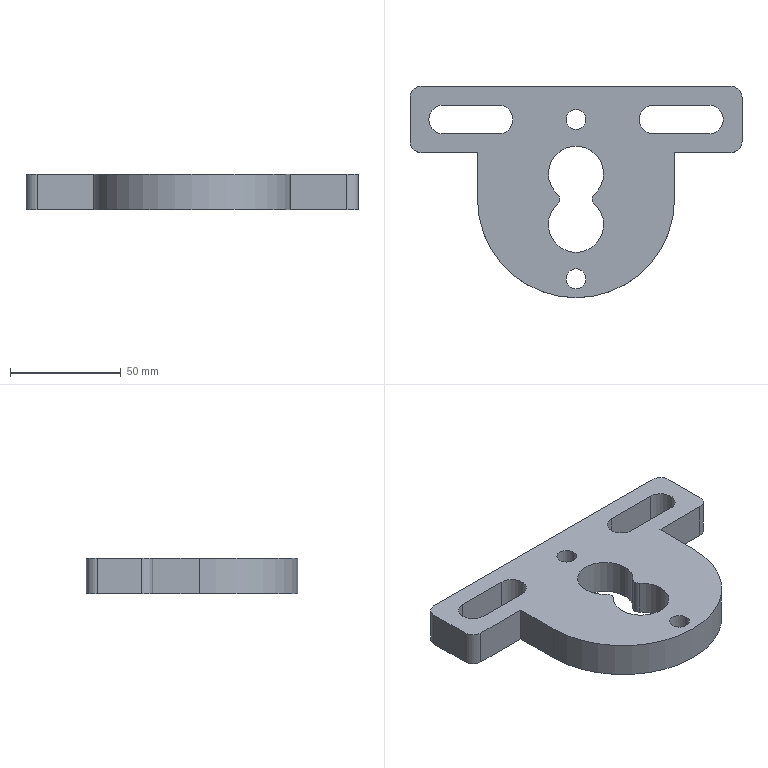Component | SolidWorks | 12AFeedInletPlate-1 | 1 solid | 43 faces | box 150 x 95.5 x 16 mm | volume 117923 mm3 | cylinder 28 | plane 15 | commonest cylinder face diameters 13 x10 25 x6 9 x4 10 x4 6 x3 89 x1 | material Q235
build123d program:
from build123d import *

# Parameters (mm, degrees)
SKETCH1_W           = 180
SKETCH1_H           = 120
BOSS_EXTRUDE1_DEPTH = 16
CUT_EXTRUDE1_DEPTH  = 110.343
CUT_EXTRUDE2_DEPTH  = 110.343
SKETCH5_R           = 4.5
CUT_EXTRUDE3_DEPTH  = 110.343
SKETCH6_R           = 6.5
CUT_EXTRUDE4_DEPTH  = 8
SKETCH7_W           = 180
SKETCH7_H           = 15
CUT_EXTRUDE5_DEPTH  = 110.343
CUT_EXTRUDE6_DEPTH  = 110.343
SKETCH9_W           = 15
SKETCH9_H           = 30
CUT_EXTRUDE7_DEPTH  = 105.433
FILLET2_R           = 5


with BuildPart() as part:
    # Sketch1 → Boss-Extrude1 (new body)
    with BuildSketch(Plane.XY):
        Rectangle(SKETCH1_W, SKETCH1_H)
    extrude(amount=BOSS_EXTRUDE1_DEPTH)

    # Sketch2 → Cut-Extrude1 (cut, through all)
    with BuildSketch(Plane.XY.offset(16)):
        with BuildLine():
            Line((-60, -23.5), (-35, -23.5))
            ThreePointArc((-35, -23.5), (-28.5, -30), (-35, -36.5))
            Line((-35, -36.5), (-60, -36.5))
            ThreePointArc((-60, -36.5), (-66.5, -30), (-60, -23.5))
        make_face()
        with BuildLine():
            Line((60, -23.5), (35, -23.5))
            ThreePointArc((35, -23.5), (28.5, -30), (35, -36.5))
            Line((35, -36.5), (60, -36.5))
            ThreePointArc((60, -36.5), (66.5, -30), (60, -23.5))
        make_face()
    extrude(amount=-CUT_EXTRUDE1_DEPTH, mode=Mode.SUBTRACT)

    # Sketch4 → Cut-Extrude2 (cut, through all)
    with BuildSketch(Plane.XY.offset(16)):
        with BuildLine():
            ThreePointArc((8.381, 8.226), (0, 30), (-8.381, 8.226))
            ThreePointArc((-8.381, 8.226), (-7.392, 6), (-8.381, 3.774))
            ThreePointArc((-8.381, 3.774), (0, -18), (8.381, 3.774))
            ThreePointArc((8.381, 3.774), (7.392, 6), (8.381, 8.226))
        make_face()
    extrude(amount=-CUT_EXTRUDE2_DEPTH, mode=Mode.SUBTRACT)

    # Sketch5 → Cut-Extrude3 (cut, through all)
    with BuildSketch(Plane.XY.offset(16)):
        with Locations((0, 42)):
            Circle(SKETCH5_R)
        with Locations(Location((0, -30, 0), (0, 0, 180))):
            Circle(SKETCH5_R)
    extrude(amount=-CUT_EXTRUDE3_DEPTH, mode=Mode.SUBTRACT)

    # Sketch6 → Cut-Extrude4 (cut)
    with BuildSketch(Plane(origin=(0, 0, 0), x_dir=(-1, 0, 0), z_dir=(0, 0, -1))):
        with Locations((0, 42)):
            Circle(SKETCH6_R)
        with Locations((0, -30)):
            Circle(SKETCH6_R)
    extrude(amount=-CUT_EXTRUDE4_DEPTH, mode=Mode.SUBTRACT)

    # Sketch7 → Cut-Extrude5 (cut, through all)
    with BuildSketch(Plane.XY.offset(16)):
        with Locations((0, -52.5)):
            Rectangle(SKETCH7_W, SKETCH7_H)
    extrude(amount=-CUT_EXTRUDE5_DEPTH, mode=Mode.SUBTRACT)

    # Sketch8 → Cut-Extrude6 (cut, through all)
    with BuildSketch(Plane.XY.offset(16)):
        with BuildLine():
            Line((-90, -15), (-44.5, -15))
            Line((-44.5, -15), (-44.5, 6))
            ThreePointArc((-44.5, 6), (0, 50.5), (44.5, 6))
            Line((44.5, 6), (44.5, -15))
            Line((44.5, -15), (90, -15))
            Line((90, -15), (90, 60))
            Line((90, 60), (50, 60))
            Line((50, 60), (-50, 60))
            Line((-50, 60), (-90, 60))
            Line((-90, 60), (-90, -15))
        make_face()
    extrude(amount=-CUT_EXTRUDE6_DEPTH, mode=Mode.SUBTRACT)

    # Sketch9 → Cut-Extrude7 (cut, through all)
    with BuildSketch(Plane.XY.offset(16)):
        with Locations((-82.5, -30)):
            Rectangle(SKETCH9_W, SKETCH9_H)
        with Locations((82.5, -30)):
            Rectangle(SKETCH9_W, SKETCH9_H)
    extrude(amount=-CUT_EXTRUDE7_DEPTH, mode=Mode.SUBTRACT)

    # Fillet2
    fillet2_edges = [part.edges().sort_by_distance(p)[0] for p in [
        (-75, -15, 8),
        (-75, -45, 8),
        (75, -45, 8),
        (75, -15, 8),
    ]]
    fillet(fillet2_edges, radius=FILLET2_R)


solid = part.part

# Placed as in the assembly
solid = solid.moved(Location((159.117, 111.71, 566), (0, 0, 180)))